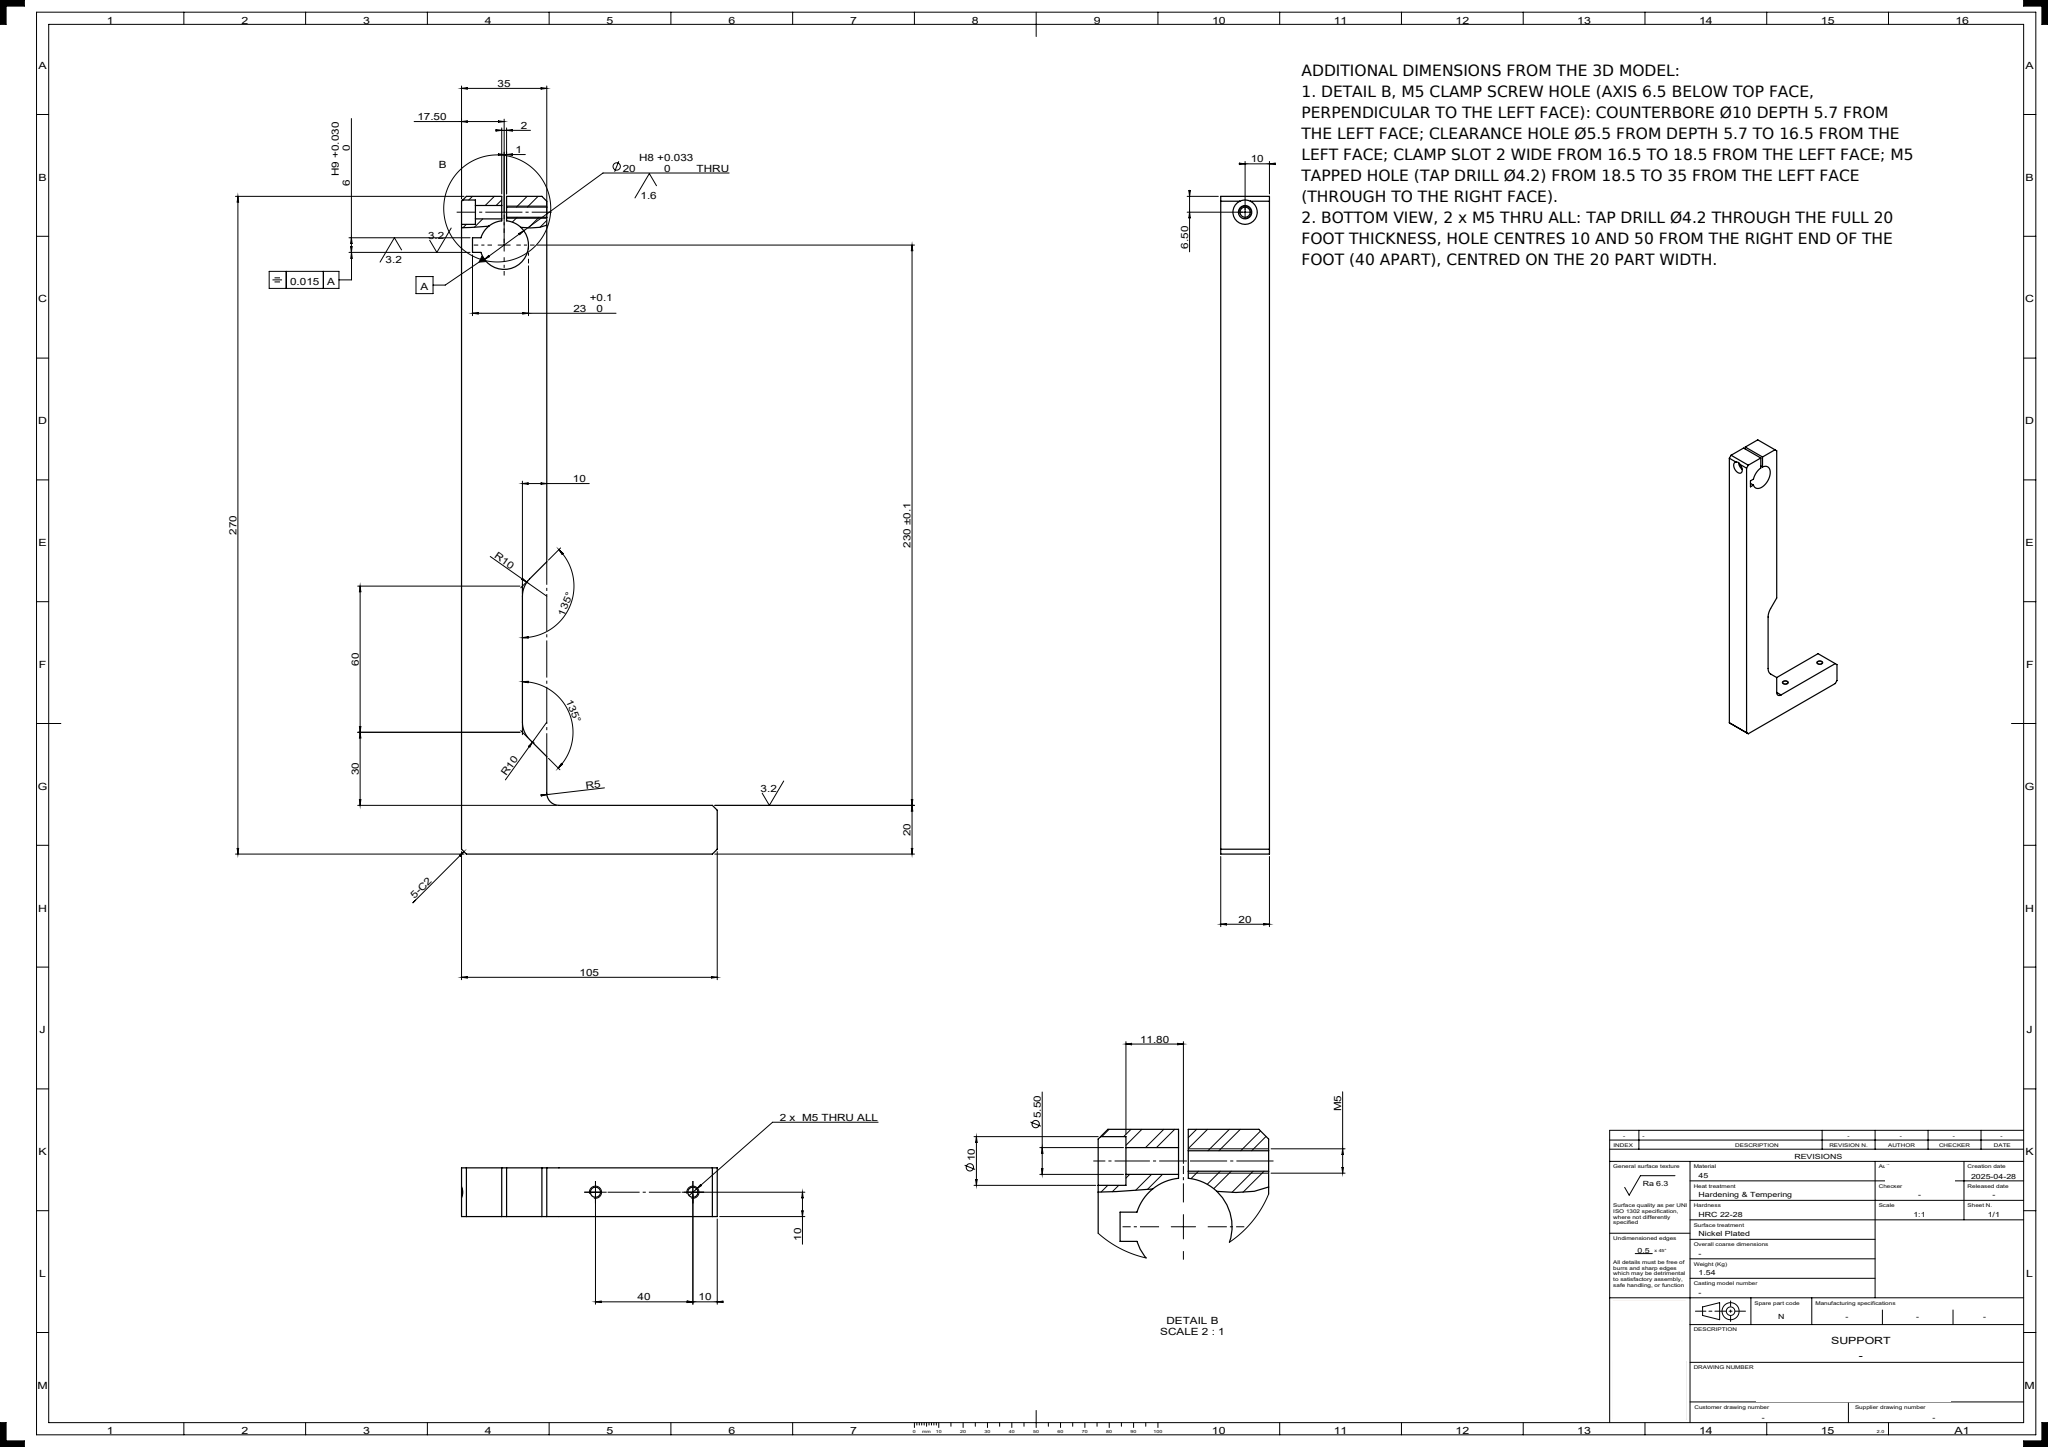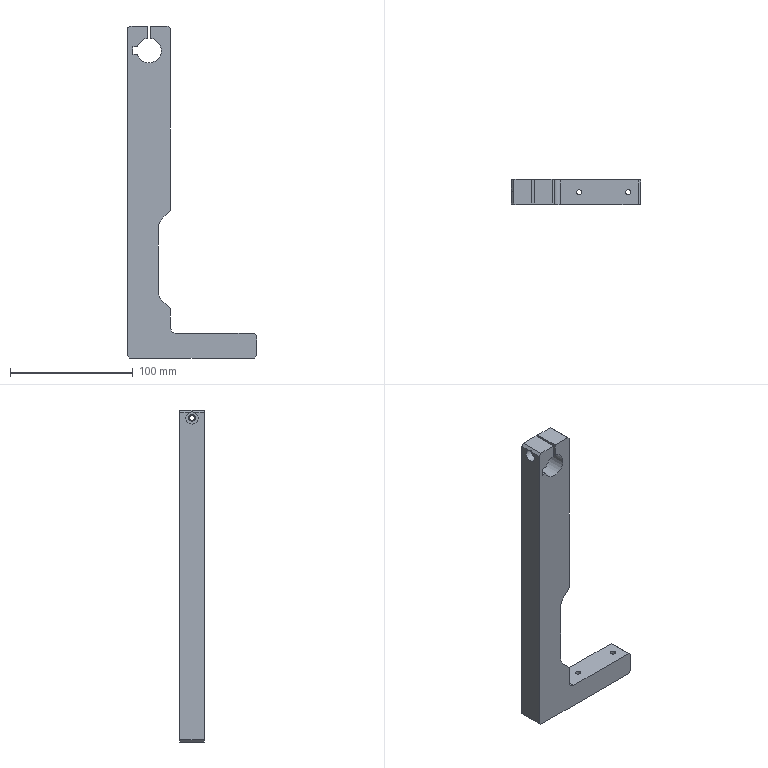Part | NX | mm | 1 solid | 34 faces | box 105 x 20 x 270 mm | volume 194445 mm3 | plane 24 | cylinder 10 | commonest cylinder face diameters 20 x4 4.2 x3 10 x2 5.5 x1